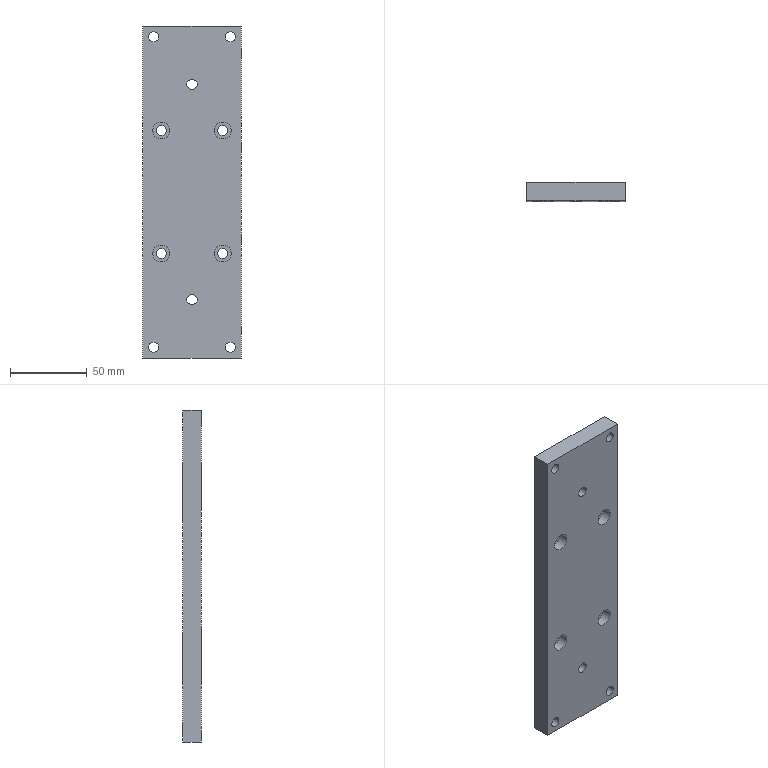Component | SolidWorks | 8TC-A15004-D0-08A-1 | 1 solid | 66 faces | box 64 x 12 x 216 mm | volume 157401 mm3 | cylinder 44 | plane 14 | cone 8 | commonest cylinder face diameters 11 x16 6.6 x16 5 x8 6.8 x4 | material #45
build123d program:
from build123d import *

# Parameters (mm, degrees)
SKETCH1_W                                       = 216
SKETCH1_H                                       = 64
BOSS_EXTRUDE1_DEPTH                             = 6
M8_TAPPED_HOLE1_D                               = 6.8
M6_HEX_SOCKET_HEAD_CAP_SCREW_CBORE1_D           = 6.6
M6_HEX_SOCKET_HEAD_CAP_SCREW_CBORE1_CBORE_D     = 11
M6_HEX_SOCKET_HEAD_CAP_SCREW_CBORE1_CBORE_DEPTH = 6.4
M6_HEX_SOCKET_HEAD_CAP_SCREW_CBORE2_D           = 6.6
M6_HEX_SOCKET_HEAD_CAP_SCREW_CBORE2_CBORE_D     = 11
M6_HEX_SOCKET_HEAD_CAP_SCREW_CBORE2_CBORE_DEPTH = 6.4
M6_TAPPED_HOLE1_D                               = 5
M6_TAPPED_HOLE1_DEPTH                           = 15
M6_TAPPED_HOLE1_TIP                             = 1.502


with BuildPart() as part:
    # Sketch1 → Boss-Extrude1 (new, symmetric)
    with BuildSketch(Plane(origin=(0, 0, 0), x_dir=(1, 0, 0), z_dir=(0, 1, 0))):
        Rectangle(SKETCH1_W, SKETCH1_H)
    extrude(amount=BOSS_EXTRUDE1_DEPTH, both=True)

    # M8 Tapped Hole1 (through all)
    with Locations(Plane(origin=(0, -6, 0), x_dir=(-1, 0, 0), z_dir=(0, -1, 0))):
        with Locations((-70, 0), (70, 0)):
            Hole(M8_TAPPED_HOLE1_D / 2)

    # M6 Hex Socket Head Cap Screw CBORE1 (through all)
    with Locations(Plane(origin=(0, -6, 0), x_dir=(-1, 0, 0), z_dir=(0, -1, 0))):
        with Locations((-101, 25), (-101, -25), (101, 25), (101, -25)):
            CounterBoreHole(M6_HEX_SOCKET_HEAD_CAP_SCREW_CBORE1_D / 2, M6_HEX_SOCKET_HEAD_CAP_SCREW_CBORE1_CBORE_D / 2, M6_HEX_SOCKET_HEAD_CAP_SCREW_CBORE1_CBORE_DEPTH)

    # M6 Hex Socket Head Cap Screw CBORE2 (through all)
    with Locations(Plane(origin=(0, 6, 0), x_dir=(1, 0, 0), z_dir=(0, 1, 0))):
        with Locations((-40, 20), (-40, -20), (40, 20), (40, -20)):
            CounterBoreHole(M6_HEX_SOCKET_HEAD_CAP_SCREW_CBORE2_D / 2, M6_HEX_SOCKET_HEAD_CAP_SCREW_CBORE2_CBORE_D / 2, M6_HEX_SOCKET_HEAD_CAP_SCREW_CBORE2_CBORE_DEPTH)

    # M6 Tapped Hole1
    with Locations(Plane(origin=(0, 0, -32), x_dir=(-1, 0, 0), z_dir=(0, 0, -1))):
        with Locations((-90, 0), (-30, 0), (30, 0), (90, 0)):
            Hole(M6_TAPPED_HOLE1_D / 2, depth=M6_TAPPED_HOLE1_DEPTH)
            with Locations((0, 0, -(M6_TAPPED_HOLE1_DEPTH + M6_TAPPED_HOLE1_TIP / 2))):  # 118° drill point
                Cone(0, M6_TAPPED_HOLE1_D / 2, M6_TAPPED_HOLE1_TIP, mode=Mode.SUBTRACT)


solid = part.part

# Placed as in the assembly
solid = solid.moved(Location((-7.5, 338.5, 0), (180, -90, 0)))